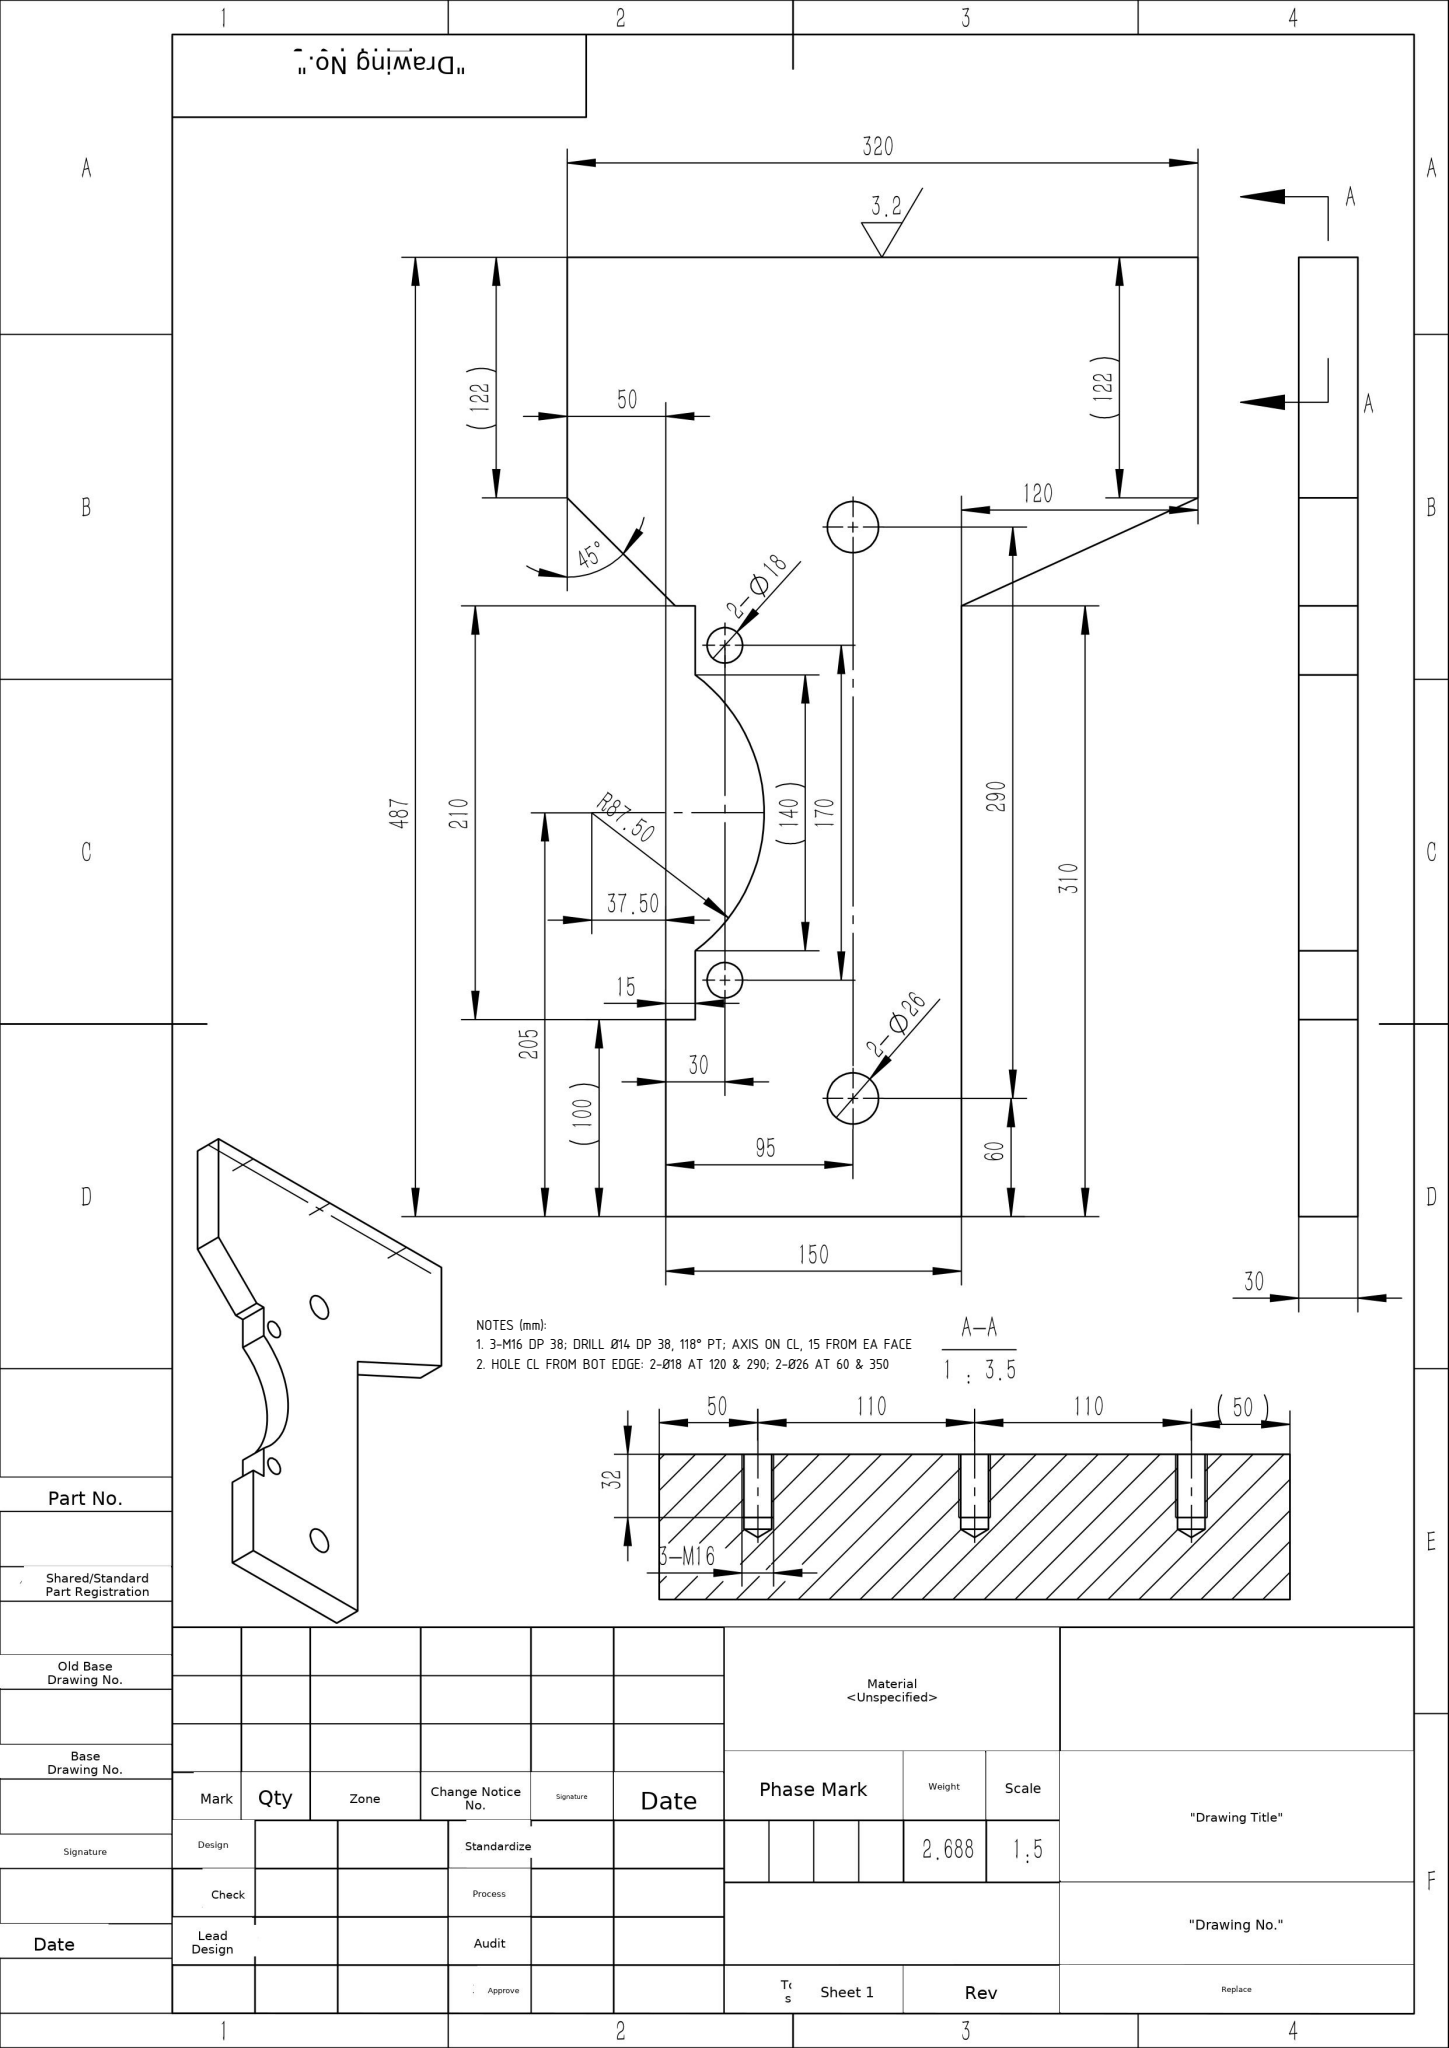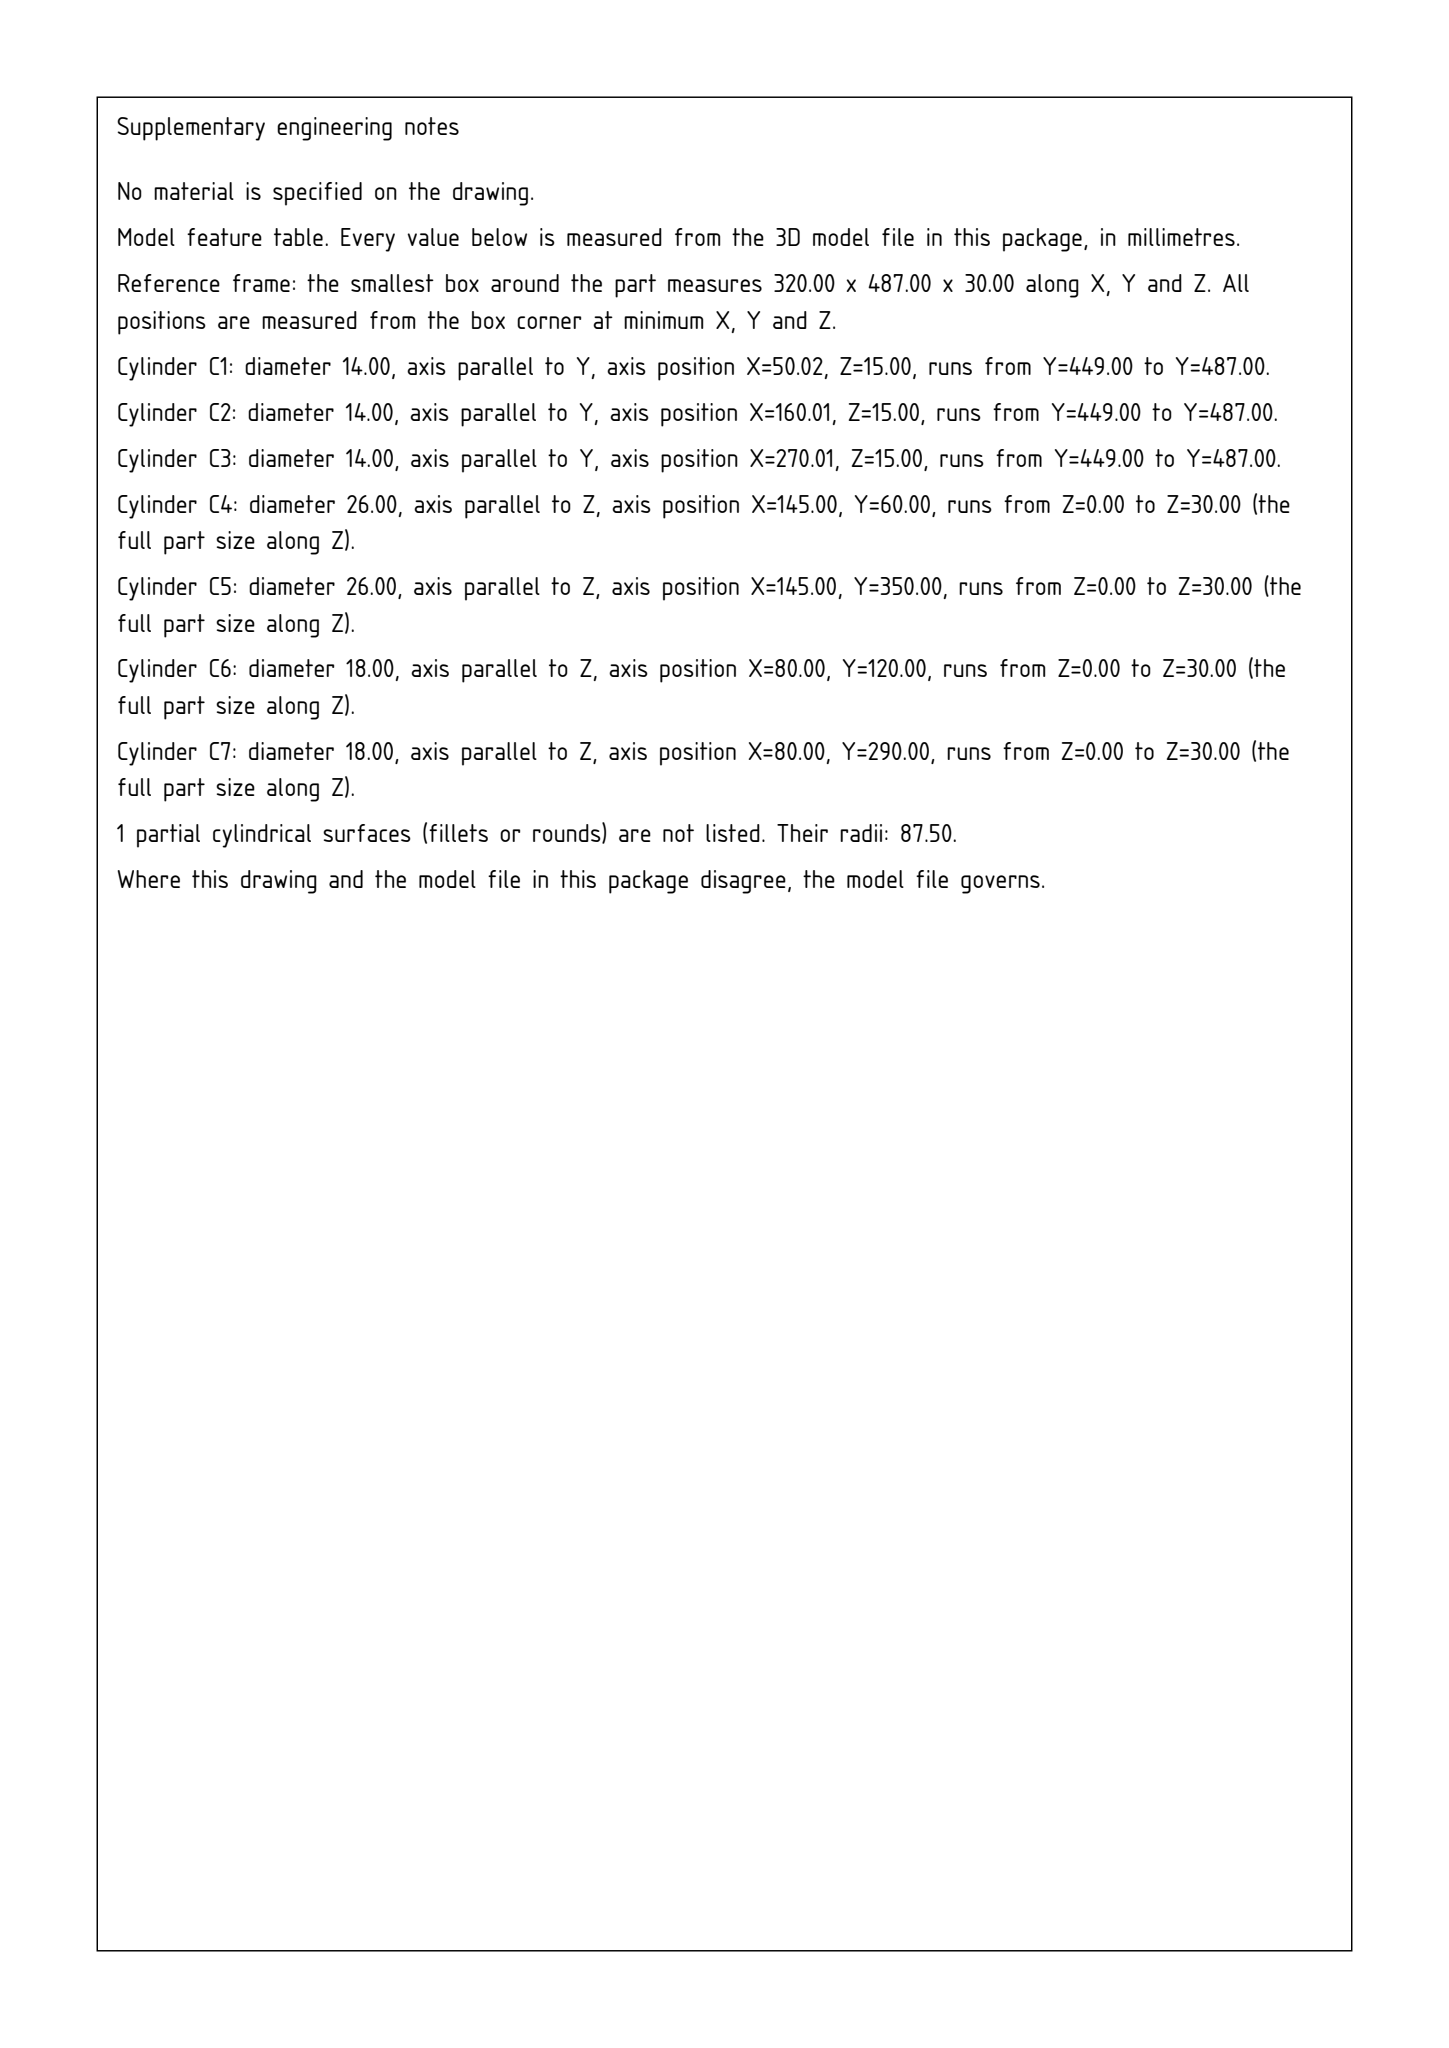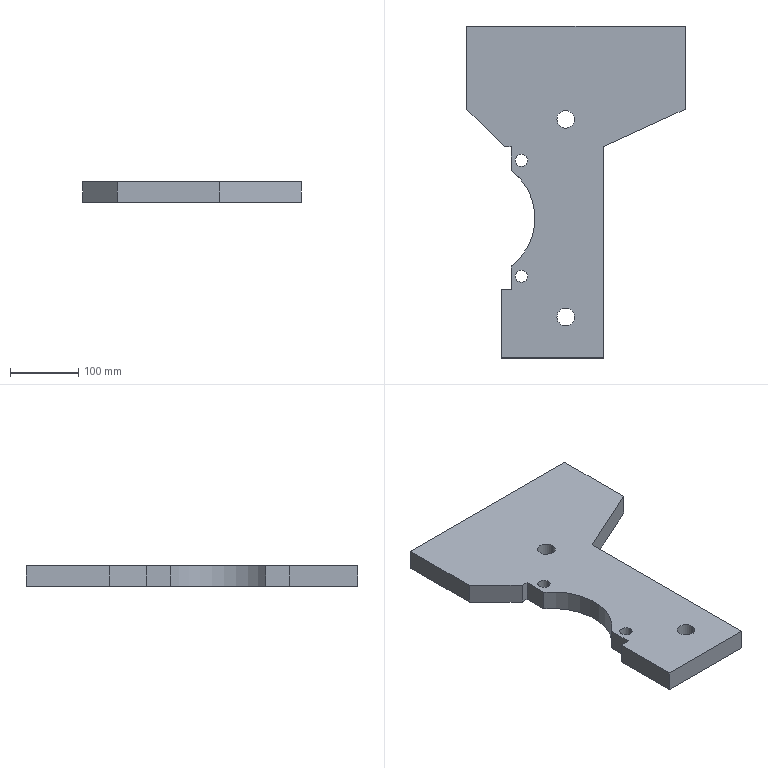Part | SolidWorks | mm | 1 solid | 35 faces | box 320 x 487 x 30 mm | volume 2687743 mm3 | cylinder 15 | plane 14 | cone 6 | commonest cylinder face diameters 14 x6 18 x4 26 x4 175 x1
Drawing notes:
3-M16 DP 38; DRILL Ø14 DP 38, 118° PT; AXIS ON CL, 15 FROM EA FACE | from the solid: Ø14 cyl axis y, L=38, pos (x,z)=(50.02,15),(160.01,15),(270.01,15); cone 118° ref dia 14, qty 3; z planes 0/30 = thk 30
HOLE CL FROM BOT EDGE: 2-Ø18 AT 120 & 290; 2-Ø26 AT 60 & 350 | from the solid: Ø18 z-holes at y=120 & 290 (x=80); Ø26 z-holes at y=60 & 350 (x=145); bbox y=487
build123d program:
from build123d import *

# Parameters (mm, degrees)
SKETCH1_R              = 13
SKETCH1_R_2            = 9
BOSS_EXTRUDE1_DEPTH    = 30
M16_TAPPED_HOLE2_D     = 14
M16_TAPPED_HOLE2_DEPTH = 38
M16_TAPPED_HOLE2_TIP   = 4.206


with BuildPart() as part:
    # Sketch1 → Boss-Extrude1 (new body)
    with BuildSketch(Plane.XY):
        with BuildLine():
            Line((0, 0), (150, 0))
            Line((150, 0), (150, 310))
            Line((150, 310), (270, 364.862))
            Line((270, 364.862), (270, 487))
            Line((270, 487), (-50, 487))
            Line((-50, 487), (-50, 364.862))
            Line((-50, 364.862), (4.862, 310))
            Line((4.862, 310), (15, 310))
            Line((15, 310), (15, 275))
            ThreePointArc((15, 275), (50, 205), (15, 135))
            Line((15, 135), (15, 100))
            Line((15, 100), (0, 100))
            Line((0, 100), (0, 0))
        make_face()
        with Locations((95, 350)):
            Circle(SKETCH1_R, mode=Mode.SUBTRACT)
        with Locations((95, 60)):
            Circle(SKETCH1_R, mode=Mode.SUBTRACT)
        with Locations((30, 290)):
            Circle(SKETCH1_R_2, mode=Mode.SUBTRACT)
        with Locations((30, 120)):
            Circle(SKETCH1_R_2, mode=Mode.SUBTRACT)
    extrude(amount=BOSS_EXTRUDE1_DEPTH)

    # M16 Tapped Hole2
    with Locations(Plane(origin=(220.008, 487, 15), x_dir=(1, 0, 0), z_dir=(0, 1, 0))):
        with Locations((0, 0), (-109.994, 0), (-219.989, 0)):
            Hole(M16_TAPPED_HOLE2_D / 2, depth=M16_TAPPED_HOLE2_DEPTH)
            with Locations((0, 0, -(M16_TAPPED_HOLE2_DEPTH + M16_TAPPED_HOLE2_TIP / 2))):  # 118° drill point
                Cone(0, M16_TAPPED_HOLE2_D / 2, M16_TAPPED_HOLE2_TIP, mode=Mode.SUBTRACT)


solid = part.part